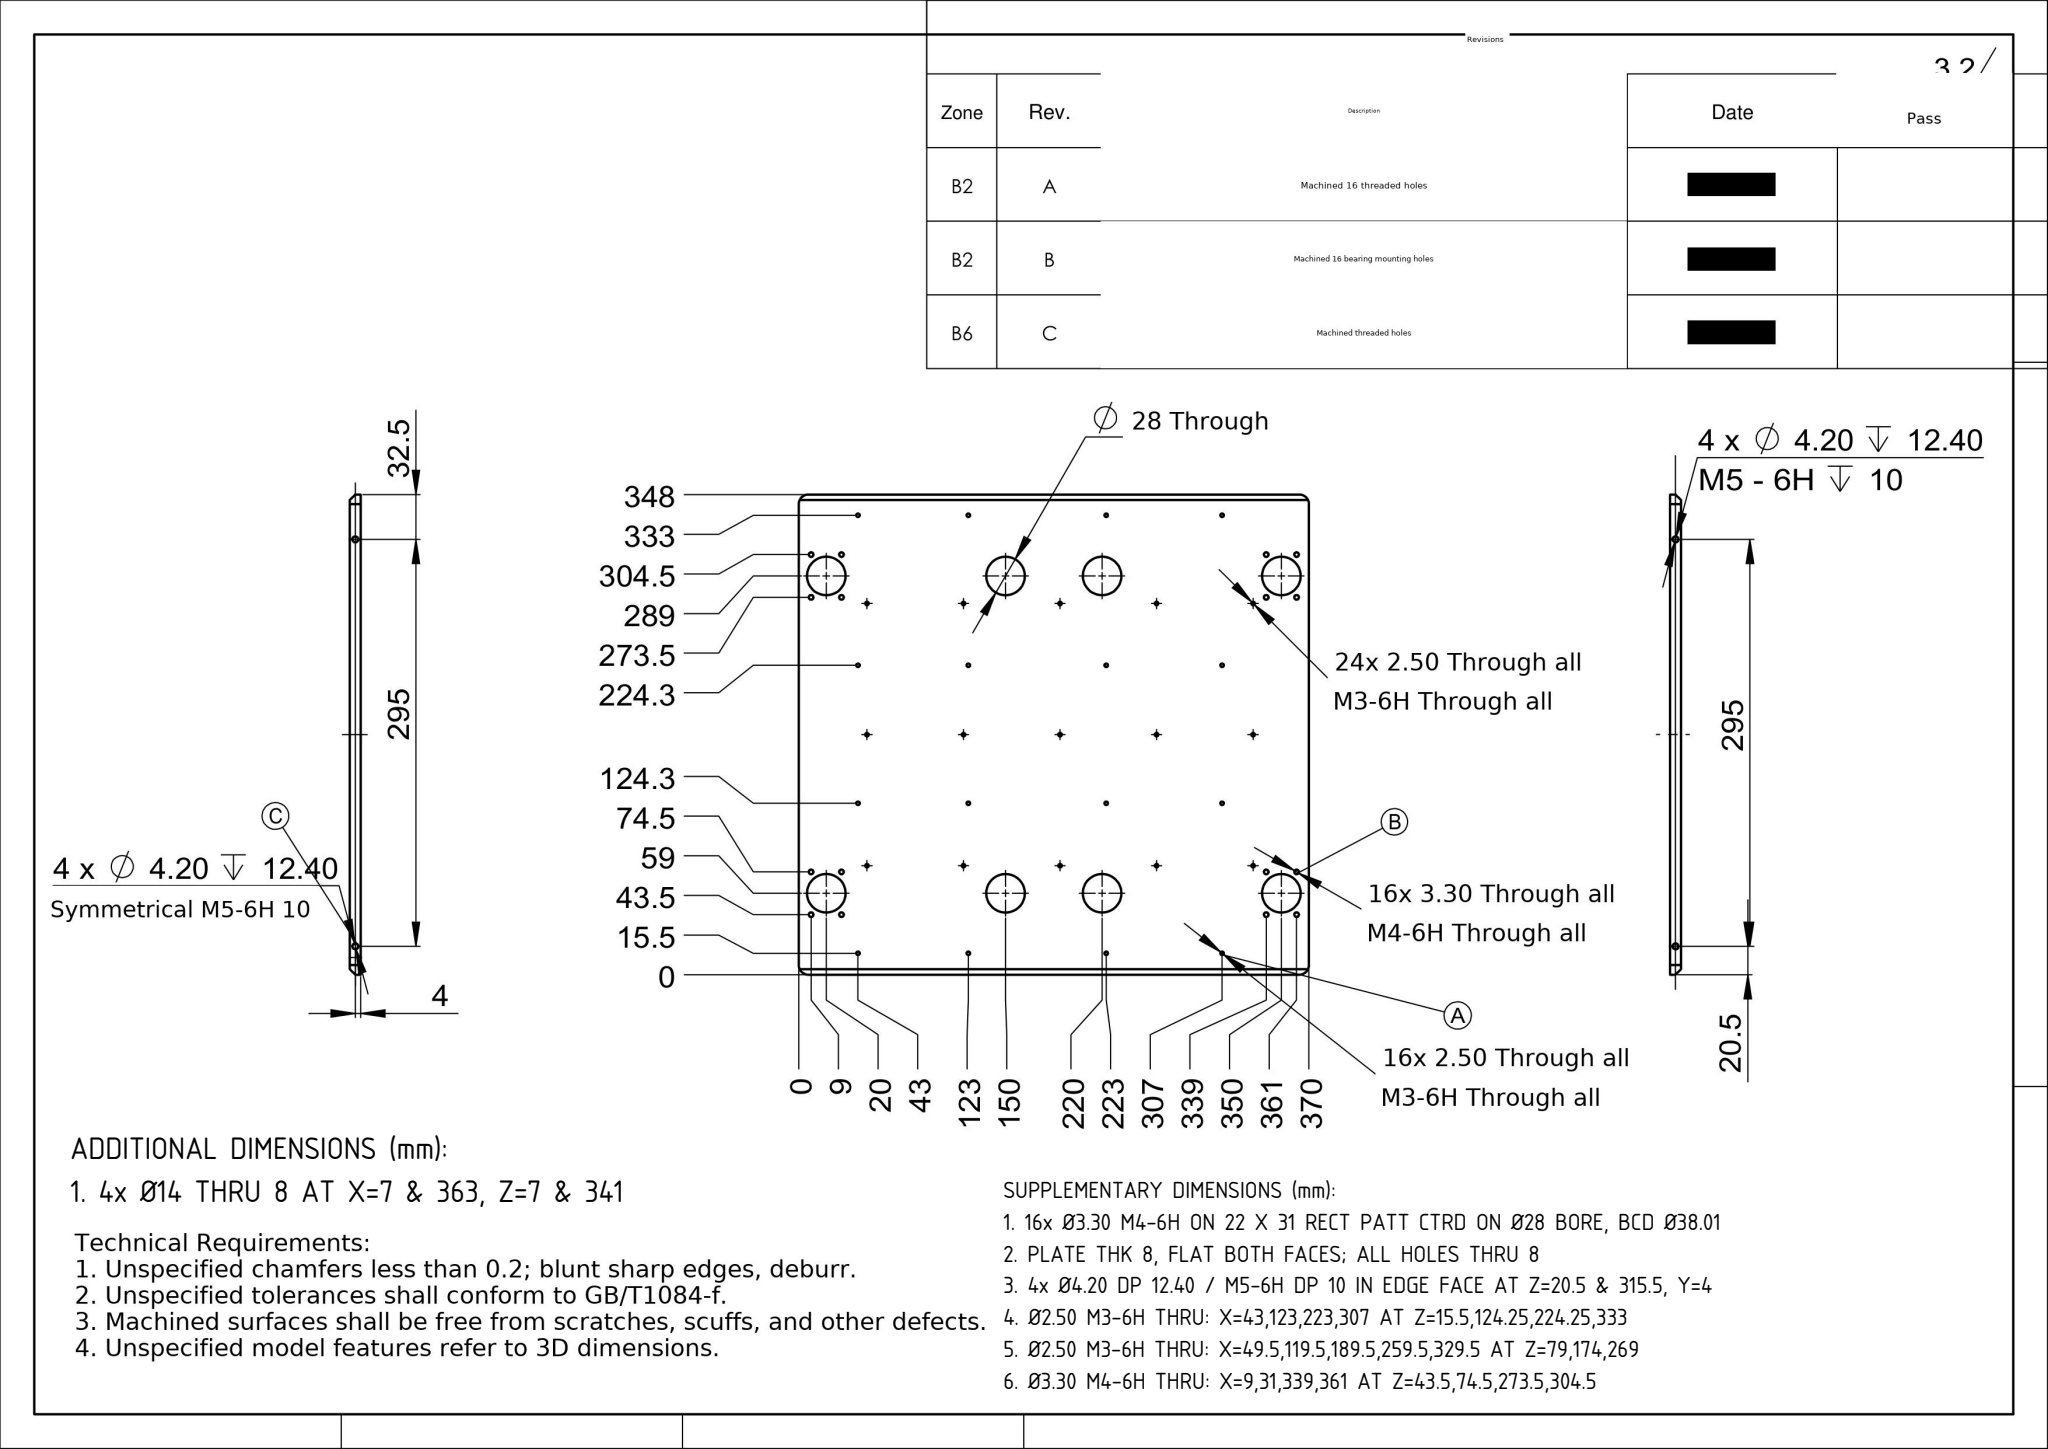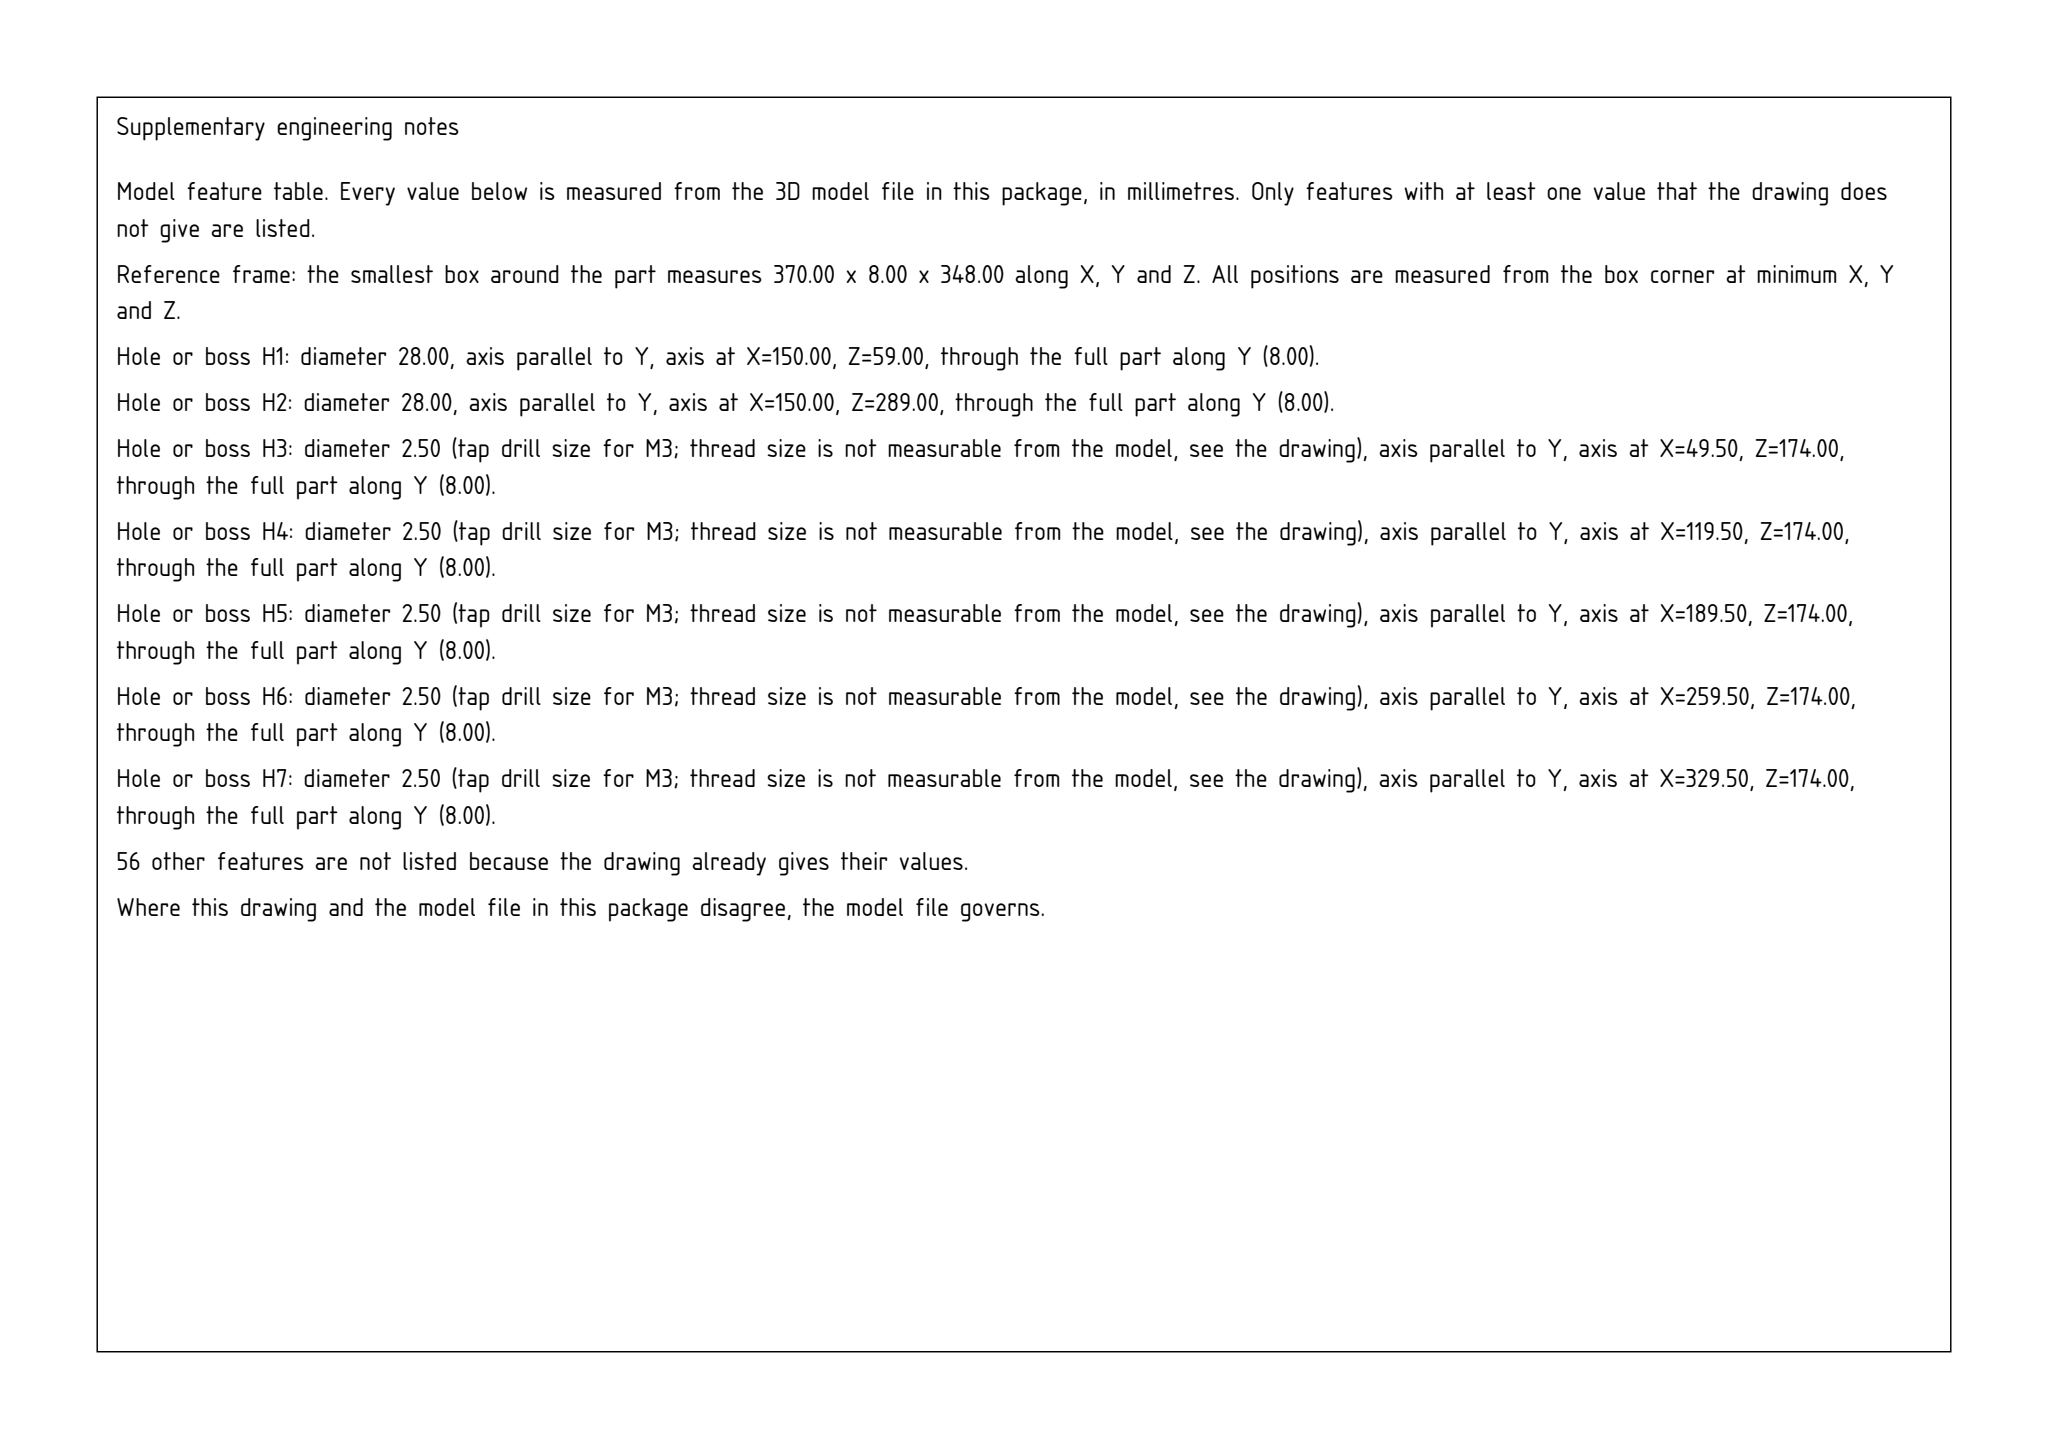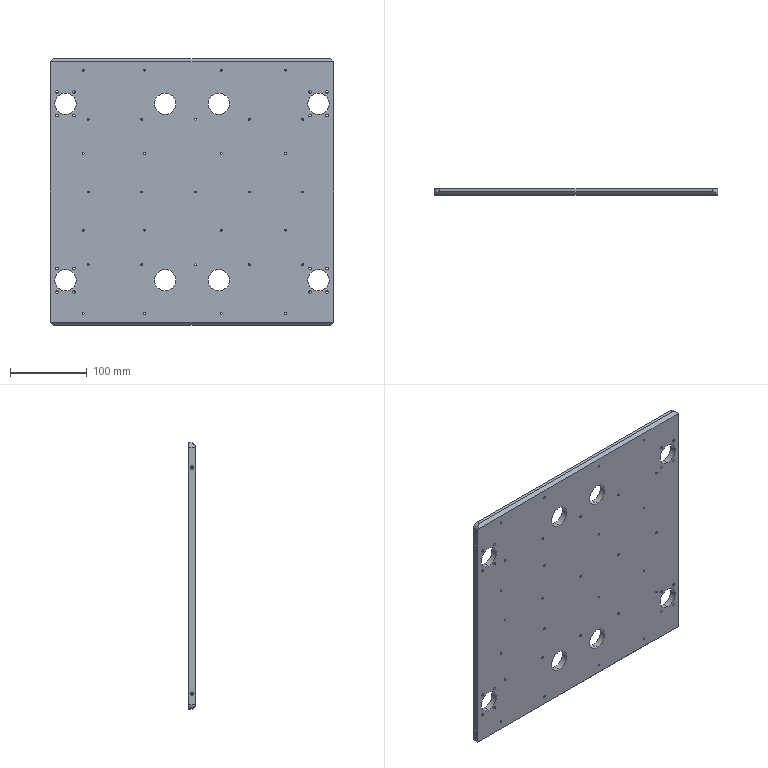Part | SolidWorks | mm | 1 solid | 138 faces | box 370 x 8 x 348 mm | volume 981497 mm3 | cylinder 122 | cone 8 | plane 8 | commonest cylinder face diameters 2.5 x62 3.3 x32 28 x16 4.2 x8 14 x4